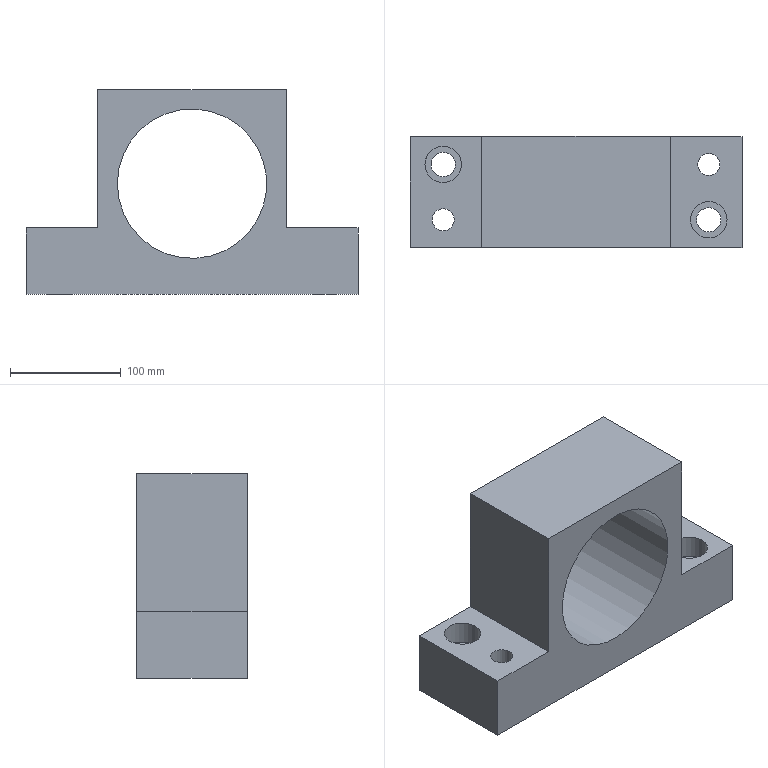Component | NX | JIG_PLATE | 1 solid | 21 faces | volume 2388298 mm3 | plane 12 | cylinder 8 | cone 1 | commonest cylinder face diameters 22 x2 33 x2 20 x2 135 x1 10 x1